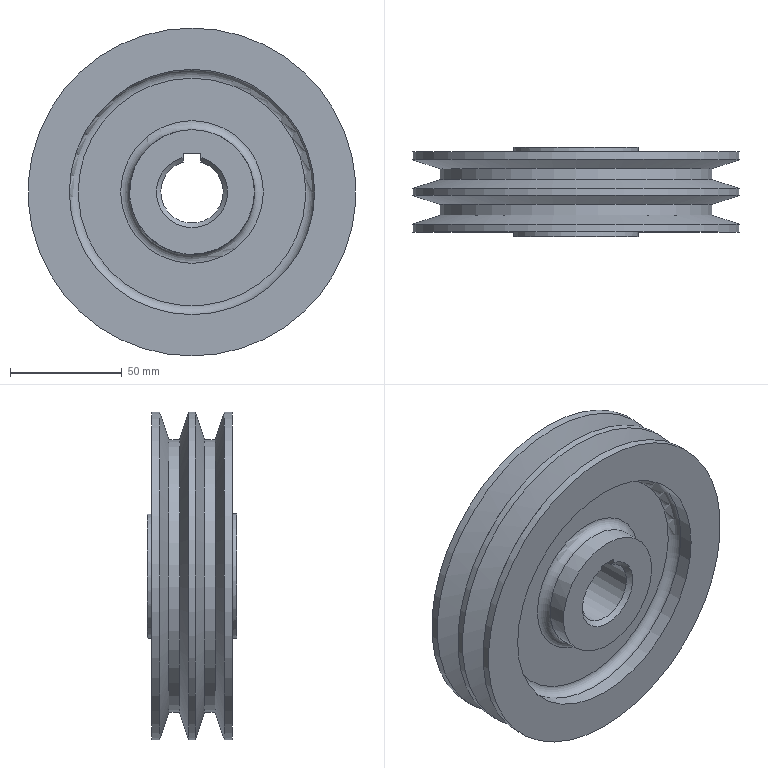Component | NX | PULLEY | 1 solid | 29 faces | volume 354731 mm3 | cylinder 10 | plane 9 | cone 6 | torus 4 | commonest cylinder face diameters 147 x3 110 x2 122 x2 56 x2 28 x1